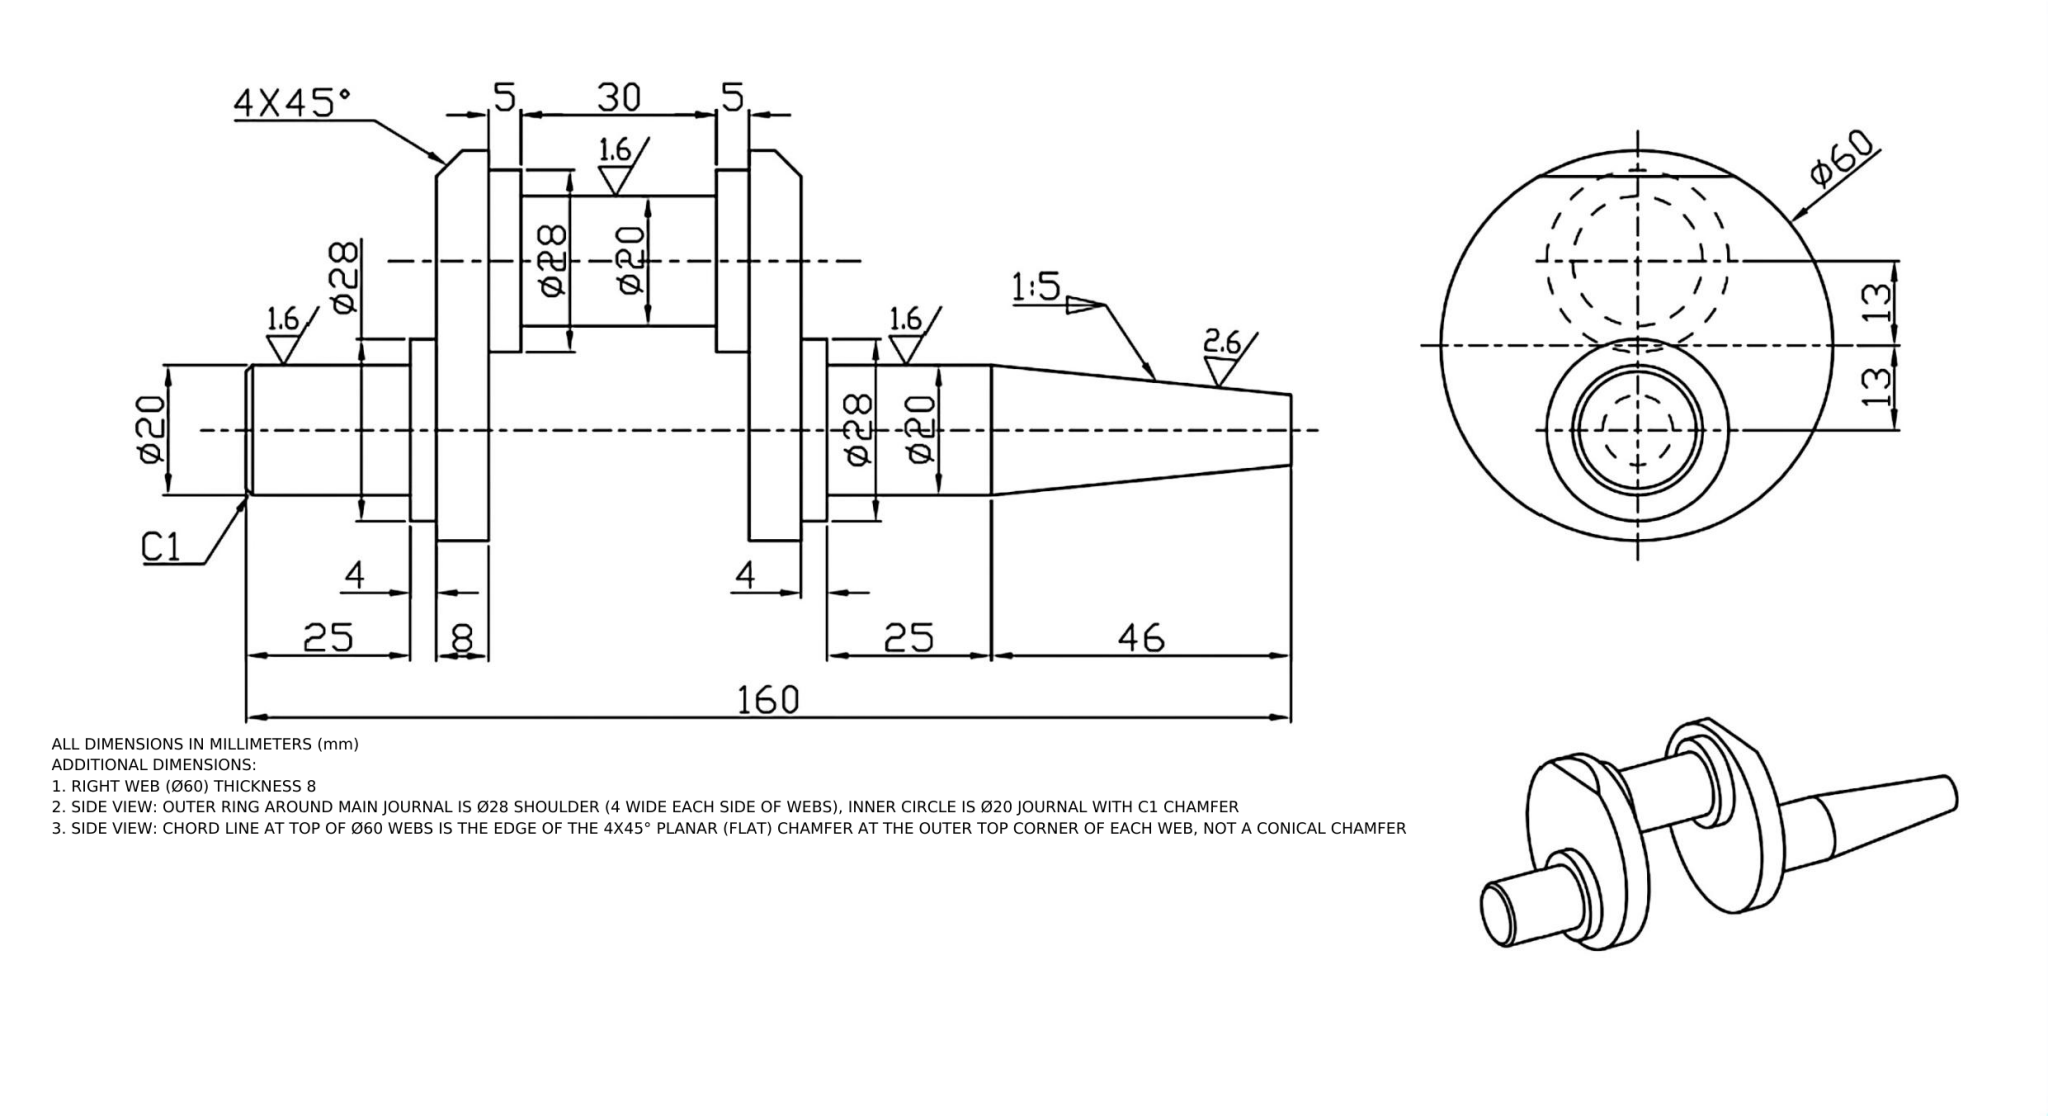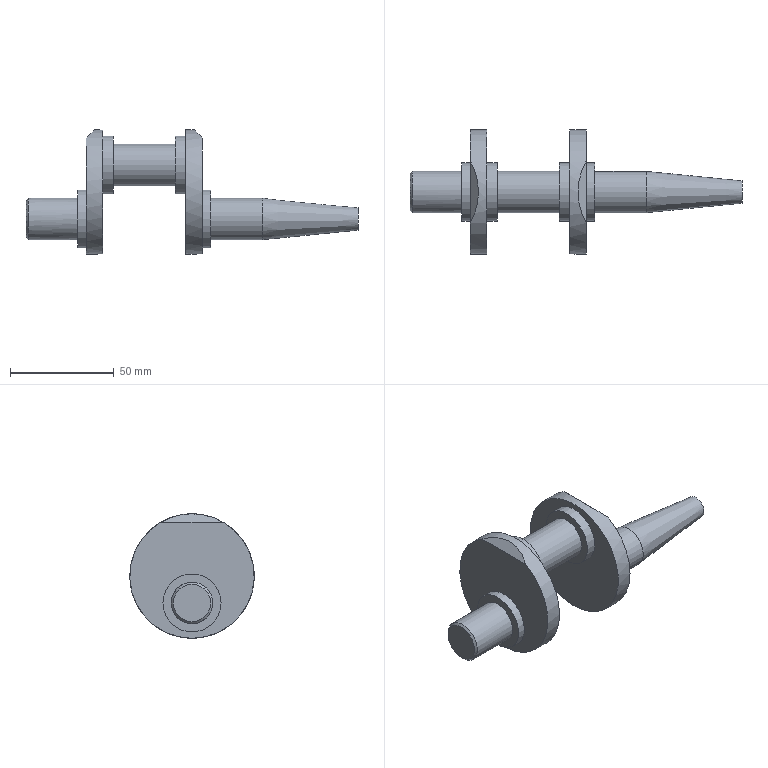Part | NX | mm | 1 solid | 23 faces | box 160 x 60 x 60 mm | volume 89987 mm3 | plane 12 | cylinder 9 | cone 2 | commonest cylinder face diameters 28 x4 20 x3 60 x2
STEP:
#1=CARTESIAN_POINT('',(0.,0.,0.));
#2=DIRECTION('',(0.,0.,1.));
#3=DIRECTION('',(1.,0.,0.));
#4=AXIS2_PLACEMENT_3D('',#1,#2,#3);
#5=(LENGTH_UNIT()NAMED_UNIT(*)SI_UNIT(.MILLI.,.METRE.));
#6=UNCERTAINTY_MEASURE_WITH_UNIT(LENGTH_MEASURE(0.00002),#5,'','');
#7=(NAMED_UNIT(*)PLANE_ANGLE_UNIT()SI_UNIT($,.RADIAN.));
#8=PLANE_ANGLE_MEASURE_WITH_UNIT(PLANE_ANGLE_MEASURE(0.01745),#7);
#9=DIMENSIONAL_EXPONENTS(0.,0.,0.,0.,0.,0.,0.);
#10=(CONVERSION_BASED_UNIT('',#8)NAMED_UNIT(#9)PLANE_ANGLE_UNIT());
#11=(NAMED_UNIT(*)SI_UNIT($,.STERADIAN.)SOLID_ANGLE_UNIT());
#12=(GEOMETRIC_REPRESENTATION_CONTEXT(3)GLOBAL_UNCERTAINTY_ASSIGNED_CONTEXT((#6))GLOBAL_UNIT_ASSIGNED_CONTEXT((#5,#10,#11))REPRESENTATION_CONTEXT('',''));
#13=SHAPE_REPRESENTATION('',(#4),#12);
#14=CARTESIAN_POINT('',(37.,30.,13.));
#15=VERTEX_POINT('',#14);
#16=CARTESIAN_POINT('',(37.,0.,13.));
#17=DIRECTION('',(1.,0.,0.));
#18=DIRECTION('',(0.,1.,-0.));
#19=AXIS2_PLACEMENT_3D('',#16,#17,#18);
#20=CIRCLE('',#19,30.);
#21=EDGE_CURVE('',#15,#15,#20,.T.);
#22=ORIENTED_EDGE('',*,*,#21,.F.);
#23=EDGE_LOOP('',(#22));
#24=FACE_BOUND('',#23,.T.);
#25=CARTESIAN_POINT('',(29.,-14.967,39.));
#26=VERTEX_POINT('',#25);
#27=CARTESIAN_POINT('',(29.,14.967,39.));
#28=VERTEX_POINT('',#27);
#29=CARTESIAN_POINT('',(3.,0.,13.));
#30=DIRECTION('',(-0.7071,0.,0.7071));
#31=DIRECTION('',(-0.7071,0.,-0.7071));
#32=AXIS2_PLACEMENT_3D('',#29,#30,#31);
#33=ELLIPSE('',#32,42.426,30.);
#34=EDGE_CURVE('',#26,#28,#33,.T.);
#35=ORIENTED_EDGE('',*,*,#34,.F.);
#36=CARTESIAN_POINT('',(29.,0.,13.));
#37=DIRECTION('',(1.,0.,0.));
#38=DIRECTION('',(0.,1.,-0.));
#39=AXIS2_PLACEMENT_3D('',#36,#37,#38);
#40=CIRCLE('',#39,30.);
#41=EDGE_CURVE('',#26,#28,#40,.T.);
#42=ORIENTED_EDGE('',*,*,#41,.T.);
#43=EDGE_LOOP('',(#35,#42));
#44=FACE_BOUND('',#43,.T.);
#45=CARTESIAN_POINT('',(37.,0.,13.));
#46=DIRECTION('',(-1.,0.,0.));
#47=DIRECTION('',(0.,0.,1.));
#48=AXIS2_PLACEMENT_3D('',#45,#46,#47);
#49=CYLINDRICAL_SURFACE('',#48,30.);
#50=ADVANCED_FACE('',(#24,#44),#49,.T.);
#51=CARTESIAN_POINT('',(1.,0.,-10.));
#52=VERTEX_POINT('',#51);
#53=CARTESIAN_POINT('',(1.,0.,0.));
#54=DIRECTION('',(1.,0.,0.));
#55=DIRECTION('',(0.,0.,-1.));
#56=AXIS2_PLACEMENT_3D('',#53,#54,#55);
#57=CIRCLE('',#56,10.);
#58=EDGE_CURVE('',#52,#52,#57,.T.);
#59=ORIENTED_EDGE('',*,*,#58,.T.);
#60=EDGE_LOOP('',(#59));
#61=FACE_BOUND('',#60,.T.);
#62=CARTESIAN_POINT('',(25.,10.,-0.));
#63=VERTEX_POINT('',#62);
#64=CARTESIAN_POINT('',(25.,0.,0.));
#65=DIRECTION('',(1.,0.,0.));
#66=DIRECTION('',(0.,1.,-0.));
#67=AXIS2_PLACEMENT_3D('',#64,#65,#66);
#68=CIRCLE('',#67,10.);
#69=EDGE_CURVE('',#63,#63,#68,.T.);
#70=ORIENTED_EDGE('',*,*,#69,.F.);
#71=EDGE_LOOP('',(#70));
#72=FACE_BOUND('',#71,.T.);
#73=CARTESIAN_POINT('',(25.,0.,0.));
#74=DIRECTION('',(-1.,0.,0.));
#75=DIRECTION('',(0.,0.,1.));
#76=AXIS2_PLACEMENT_3D('',#73,#74,#75);
#77=CYLINDRICAL_SURFACE('',#76,10.);
#78=ADVANCED_FACE('',(#61,#72),#77,.T.);
#79=CARTESIAN_POINT('',(0.,0.,-9.));
#80=VERTEX_POINT('',#79);
#81=CARTESIAN_POINT('',(0.,0.,0.));
#82=DIRECTION('',(-1.,0.,0.));
#83=DIRECTION('',(0.,0.,-1.));
#84=AXIS2_PLACEMENT_3D('',#81,#82,#83);
#85=CIRCLE('',#84,9.);
#86=EDGE_CURVE('',#80,#80,#85,.T.);
#87=ORIENTED_EDGE('',*,*,#86,.T.);
#88=EDGE_LOOP('',(#87));
#89=FACE_OUTER_BOUND('',#88,.T.);
#90=CARTESIAN_POINT('',(0.,0.,0.));
#91=DIRECTION('',(1.,0.,0.));
#92=DIRECTION('',(0.,0.,-1.));
#93=AXIS2_PLACEMENT_3D('',#90,#91,#92);
#94=PLANE('',#93);
#95=ADVANCED_FACE('',(#89),#94,.F.);
#96=ORIENTED_EDGE('',*,*,#86,.F.);
#97=EDGE_LOOP('',(#96));
#98=FACE_BOUND('',#97,.T.);
#99=ORIENTED_EDGE('',*,*,#58,.F.);
#100=EDGE_LOOP('',(#99));
#101=FACE_BOUND('',#100,.T.);
#102=CARTESIAN_POINT('',(1.,0.,0.));
#103=DIRECTION('',(1.,0.,0.));
#104=DIRECTION('',(-0.,0.,-1.));
#105=AXIS2_PLACEMENT_3D('',#102,#103,#104);
#106=CONICAL_SURFACE('',#105,10.,45.);
#107=ADVANCED_FACE('',(#98,#101),#106,.T.);
#108=CARTESIAN_POINT('',(37.,14.,26.));
#109=VERTEX_POINT('',#108);
#110=CARTESIAN_POINT('',(37.,0.,26.));
#111=DIRECTION('',(1.,0.,0.));
#112=DIRECTION('',(0.,1.,0.));
#113=AXIS2_PLACEMENT_3D('',#110,#111,#112);
#114=CIRCLE('',#113,14.);
#115=EDGE_CURVE('',#109,#109,#114,.T.);
#116=ORIENTED_EDGE('',*,*,#115,.F.);
#117=EDGE_LOOP('',(#116));
#118=FACE_BOUND('',#117,.T.);
#119=ORIENTED_EDGE('',*,*,#21,.T.);
#120=EDGE_LOOP('',(#119));
#121=FACE_BOUND('',#120,.T.);
#122=CARTESIAN_POINT('',(37.,0.,13.));
#123=DIRECTION('',(1.,0.,0.));
#124=DIRECTION('',(0.,0.,-1.));
#125=AXIS2_PLACEMENT_3D('',#122,#123,#124);
#126=PLANE('',#125);
#127=ADVANCED_FACE('',(#118,#121),#126,.T.);
#128=CARTESIAN_POINT('',(29.,14.,-0.));
#129=VERTEX_POINT('',#128);
#130=CARTESIAN_POINT('',(29.,0.,0.));
#131=DIRECTION('',(1.,0.,0.));
#132=DIRECTION('',(0.,1.,-0.));
#133=AXIS2_PLACEMENT_3D('',#130,#131,#132);
#134=CIRCLE('',#133,14.);
#135=EDGE_CURVE('',#129,#129,#134,.T.);
#136=ORIENTED_EDGE('',*,*,#135,.T.);
#137=EDGE_LOOP('',(#136));
#138=FACE_BOUND('',#137,.T.);
#139=ORIENTED_EDGE('',*,*,#41,.F.);
#140=CARTESIAN_POINT('',(29.,-47.,39.));
#141=DIRECTION('',(0.,1.,0.));
#142=VECTOR('',#141,1.);
#143=LINE('',#140,#142);
#144=EDGE_CURVE('',#26,#28,#143,.T.);
#145=ORIENTED_EDGE('',*,*,#144,.T.);
#146=EDGE_LOOP('',(#139,#145));
#147=FACE_BOUND('',#146,.T.);
#148=CARTESIAN_POINT('',(29.,0.,13.));
#149=DIRECTION('',(1.,0.,0.));
#150=DIRECTION('',(0.,0.,-1.));
#151=AXIS2_PLACEMENT_3D('',#148,#149,#150);
#152=PLANE('',#151);
#153=ADVANCED_FACE('',(#138,#147),#152,.F.);
#154=CARTESIAN_POINT('',(42.,14.,26.));
#155=VERTEX_POINT('',#154);
#156=CARTESIAN_POINT('',(42.,0.,26.));
#157=DIRECTION('',(1.,0.,0.));
#158=DIRECTION('',(0.,1.,0.));
#159=AXIS2_PLACEMENT_3D('',#156,#157,#158);
#160=CIRCLE('',#159,14.);
#161=EDGE_CURVE('',#155,#155,#160,.T.);
#162=ORIENTED_EDGE('',*,*,#161,.F.);
#163=EDGE_LOOP('',(#162));
#164=FACE_BOUND('',#163,.T.);
#165=ORIENTED_EDGE('',*,*,#115,.T.);
#166=EDGE_LOOP('',(#165));
#167=FACE_BOUND('',#166,.T.);
#168=CARTESIAN_POINT('',(42.,0.,26.));
#169=DIRECTION('',(-1.,0.,0.));
#170=DIRECTION('',(0.,0.,1.));
#171=AXIS2_PLACEMENT_3D('',#168,#169,#170);
#172=CYLINDRICAL_SURFACE('',#171,14.);
#173=ADVANCED_FACE('',(#164,#167),#172,.T.);
#174=CARTESIAN_POINT('',(42.,10.,26.));
#175=VERTEX_POINT('',#174);
#176=CARTESIAN_POINT('',(42.,0.,26.));
#177=DIRECTION('',(1.,0.,0.));
#178=DIRECTION('',(0.,1.,0.));
#179=AXIS2_PLACEMENT_3D('',#176,#177,#178);
#180=CIRCLE('',#179,10.);
#181=EDGE_CURVE('',#175,#175,#180,.T.);
#182=ORIENTED_EDGE('',*,*,#181,.F.);
#183=EDGE_LOOP('',(#182));
#184=FACE_BOUND('',#183,.T.);
#185=ORIENTED_EDGE('',*,*,#161,.T.);
#186=EDGE_LOOP('',(#185));
#187=FACE_BOUND('',#186,.T.);
#188=CARTESIAN_POINT('',(42.,0.,26.));
#189=DIRECTION('',(1.,0.,0.));
#190=DIRECTION('',(0.,0.,-1.));
#191=AXIS2_PLACEMENT_3D('',#188,#189,#190);
#192=PLANE('',#191);
#193=ADVANCED_FACE('',(#184,#187),#192,.T.);
#194=CARTESIAN_POINT('',(72.,10.,26.));
#195=VERTEX_POINT('',#194);
#196=CARTESIAN_POINT('',(72.,0.,26.));
#197=DIRECTION('',(1.,0.,0.));
#198=DIRECTION('',(0.,1.,0.));
#199=AXIS2_PLACEMENT_3D('',#196,#197,#198);
#200=CIRCLE('',#199,10.);
#201=EDGE_CURVE('',#195,#195,#200,.T.);
#202=ORIENTED_EDGE('',*,*,#201,.F.);
#203=EDGE_LOOP('',(#202));
#204=FACE_BOUND('',#203,.T.);
#205=ORIENTED_EDGE('',*,*,#181,.T.);
#206=EDGE_LOOP('',(#205));
#207=FACE_BOUND('',#206,.T.);
#208=CARTESIAN_POINT('',(72.,0.,26.));
#209=DIRECTION('',(-1.,0.,0.));
#210=DIRECTION('',(0.,0.,1.));
#211=AXIS2_PLACEMENT_3D('',#208,#209,#210);
#212=CYLINDRICAL_SURFACE('',#211,10.);
#213=ADVANCED_FACE('',(#204,#207),#212,.T.);
#214=CARTESIAN_POINT('',(85.,14.967,39.));
#215=VERTEX_POINT('',#214);
#216=CARTESIAN_POINT('',(85.,-14.967,39.));
#217=VERTEX_POINT('',#216);
#218=CARTESIAN_POINT('',(111.,0.,13.));
#219=DIRECTION('',(0.7071,0.,0.7071));
#220=DIRECTION('',(0.7071,0.,-0.7071));
#221=AXIS2_PLACEMENT_3D('',#218,#219,#220);
#222=ELLIPSE('',#221,42.426,30.);
#223=EDGE_CURVE('',#215,#217,#222,.T.);
#224=ORIENTED_EDGE('',*,*,#223,.F.);
#225=CARTESIAN_POINT('',(85.,0.,13.));
#226=DIRECTION('',(1.,0.,0.));
#227=DIRECTION('',(0.,1.,-0.));
#228=AXIS2_PLACEMENT_3D('',#225,#226,#227);
#229=CIRCLE('',#228,30.);
#230=EDGE_CURVE('',#217,#215,#229,.T.);
#231=ORIENTED_EDGE('',*,*,#230,.F.);
#232=EDGE_LOOP('',(#224,#231));
#233=FACE_BOUND('',#232,.T.);
#234=CARTESIAN_POINT('',(77.,30.,13.));
#235=VERTEX_POINT('',#234);
#236=CARTESIAN_POINT('',(77.,0.,13.));
#237=DIRECTION('',(1.,0.,0.));
#238=DIRECTION('',(0.,1.,-0.));
#239=AXIS2_PLACEMENT_3D('',#236,#237,#238);
#240=CIRCLE('',#239,30.);
#241=EDGE_CURVE('',#235,#235,#240,.T.);
#242=ORIENTED_EDGE('',*,*,#241,.T.);
#243=EDGE_LOOP('',(#242));
#244=FACE_BOUND('',#243,.T.);
#245=CARTESIAN_POINT('',(77.,0.,13.));
#246=DIRECTION('',(1.,0.,0.));
#247=DIRECTION('',(0.,0.,-1.));
#248=AXIS2_PLACEMENT_3D('',#245,#246,#247);
#249=CYLINDRICAL_SURFACE('',#248,30.);
#250=ADVANCED_FACE('',(#233,#244),#249,.T.);
#251=CARTESIAN_POINT('',(77.,14.,26.));
#252=VERTEX_POINT('',#251);
#253=CARTESIAN_POINT('',(77.,0.,26.));
#254=DIRECTION('',(1.,0.,0.));
#255=DIRECTION('',(0.,1.,0.));
#256=AXIS2_PLACEMENT_3D('',#253,#254,#255);
#257=CIRCLE('',#256,14.);
#258=EDGE_CURVE('',#252,#252,#257,.T.);
#259=ORIENTED_EDGE('',*,*,#258,.T.);
#260=EDGE_LOOP('',(#259));
#261=FACE_BOUND('',#260,.T.);
#262=ORIENTED_EDGE('',*,*,#241,.F.);
#263=EDGE_LOOP('',(#262));
#264=FACE_BOUND('',#263,.T.);
#265=CARTESIAN_POINT('',(77.,0.,13.));
#266=DIRECTION('',(1.,0.,0.));
#267=DIRECTION('',(0.,0.,-1.));
#268=AXIS2_PLACEMENT_3D('',#265,#266,#267);
#269=PLANE('',#268);
#270=ADVANCED_FACE('',(#261,#264),#269,.F.);
#271=CARTESIAN_POINT('',(85.,-47.,39.));
#272=DIRECTION('',(0.,1.,0.));
#273=VECTOR('',#272,1.);
#274=LINE('',#271,#273);
#275=EDGE_CURVE('',#217,#215,#274,.T.);
#276=ORIENTED_EDGE('',*,*,#275,.F.);
#277=ORIENTED_EDGE('',*,*,#230,.T.);
#278=EDGE_LOOP('',(#276,#277));
#279=FACE_BOUND('',#278,.T.);
#280=CARTESIAN_POINT('',(85.,14.,-0.));
#281=VERTEX_POINT('',#280);
#282=CARTESIAN_POINT('',(85.,0.,0.));
#283=DIRECTION('',(1.,0.,0.));
#284=DIRECTION('',(0.,1.,-0.));
#285=AXIS2_PLACEMENT_3D('',#282,#283,#284);
#286=CIRCLE('',#285,14.);
#287=EDGE_CURVE('',#281,#281,#286,.T.);
#288=ORIENTED_EDGE('',*,*,#287,.F.);
#289=EDGE_LOOP('',(#288));
#290=FACE_BOUND('',#289,.T.);
#291=CARTESIAN_POINT('',(85.,0.,13.));
#292=DIRECTION('',(1.,0.,0.));
#293=DIRECTION('',(0.,0.,-1.));
#294=AXIS2_PLACEMENT_3D('',#291,#292,#293);
#295=PLANE('',#294);
#296=ADVANCED_FACE('',(#279,#290),#295,.T.);
#297=CARTESIAN_POINT('',(72.,14.,26.));
#298=VERTEX_POINT('',#297);
#299=CARTESIAN_POINT('',(72.,0.,26.));
#300=DIRECTION('',(1.,0.,0.));
#301=DIRECTION('',(0.,1.,0.));
#302=AXIS2_PLACEMENT_3D('',#299,#300,#301);
#303=CIRCLE('',#302,14.);
#304=EDGE_CURVE('',#298,#298,#303,.T.);
#305=ORIENTED_EDGE('',*,*,#304,.T.);
#306=EDGE_LOOP('',(#305));
#307=FACE_BOUND('',#306,.T.);
#308=ORIENTED_EDGE('',*,*,#258,.F.);
#309=EDGE_LOOP('',(#308));
#310=FACE_BOUND('',#309,.T.);
#311=CARTESIAN_POINT('',(72.,0.,26.));
#312=DIRECTION('',(1.,0.,0.));
#313=DIRECTION('',(0.,0.,-1.));
#314=AXIS2_PLACEMENT_3D('',#311,#312,#313);
#315=CYLINDRICAL_SURFACE('',#314,14.);
#316=ADVANCED_FACE('',(#307,#310),#315,.T.);
#317=ORIENTED_EDGE('',*,*,#201,.T.);
#318=EDGE_LOOP('',(#317));
#319=FACE_BOUND('',#318,.T.);
#320=ORIENTED_EDGE('',*,*,#304,.F.);
#321=EDGE_LOOP('',(#320));
#322=FACE_BOUND('',#321,.T.);
#323=CARTESIAN_POINT('',(72.,0.,26.));
#324=DIRECTION('',(1.,0.,0.));
#325=DIRECTION('',(0.,0.,-1.));
#326=AXIS2_PLACEMENT_3D('',#323,#324,#325);
#327=PLANE('',#326);
#328=ADVANCED_FACE('',(#319,#322),#327,.F.);
#329=ORIENTED_EDGE('',*,*,#287,.T.);
#330=EDGE_LOOP('',(#329));
#331=FACE_BOUND('',#330,.T.);
#332=CARTESIAN_POINT('',(89.,14.,-0.));
#333=VERTEX_POINT('',#332);
#334=CARTESIAN_POINT('',(89.,0.,0.));
#335=DIRECTION('',(1.,0.,0.));
#336=DIRECTION('',(0.,1.,-0.));
#337=AXIS2_PLACEMENT_3D('',#334,#335,#336);
#338=CIRCLE('',#337,14.);
#339=EDGE_CURVE('',#333,#333,#338,.T.);
#340=ORIENTED_EDGE('',*,*,#339,.F.);
#341=EDGE_LOOP('',(#340));
#342=FACE_BOUND('',#341,.T.);
#343=CARTESIAN_POINT('',(85.,0.,0.));
#344=DIRECTION('',(1.,0.,0.));
#345=DIRECTION('',(0.,0.,-1.));
#346=AXIS2_PLACEMENT_3D('',#343,#344,#345);
#347=CYLINDRICAL_SURFACE('',#346,14.);
#348=ADVANCED_FACE('',(#331,#342),#347,.T.);
#349=CARTESIAN_POINT('',(89.,0.,-10.));
#350=VERTEX_POINT('',#349);
#351=CARTESIAN_POINT('',(89.,0.,-0.));
#352=DIRECTION('',(1.,0.,0.));
#353=DIRECTION('',(0.,0.,-1.));
#354=AXIS2_PLACEMENT_3D('',#351,#352,#353);
#355=CIRCLE('',#354,10.);
#356=EDGE_CURVE('',#350,#350,#355,.T.);
#357=ORIENTED_EDGE('',*,*,#356,.F.);
#358=EDGE_LOOP('',(#357));
#359=FACE_BOUND('',#358,.T.);
#360=ORIENTED_EDGE('',*,*,#339,.T.);
#361=EDGE_LOOP('',(#360));
#362=FACE_BOUND('',#361,.T.);
#363=CARTESIAN_POINT('',(89.,0.,0.));
#364=DIRECTION('',(1.,0.,0.));
#365=DIRECTION('',(0.,0.,-1.));
#366=AXIS2_PLACEMENT_3D('',#363,#364,#365);
#367=PLANE('',#366);
#368=ADVANCED_FACE('',(#359,#362),#367,.T.);
#369=CARTESIAN_POINT('',(160.,0.,-5.4));
#370=VERTEX_POINT('',#369);
#371=CARTESIAN_POINT('',(160.,0.,0.));
#372=DIRECTION('',(1.,0.,0.));
#373=DIRECTION('',(0.,0.,-1.));
#374=AXIS2_PLACEMENT_3D('',#371,#372,#373);
#375=CIRCLE('',#374,5.4);
#376=EDGE_CURVE('',#370,#370,#375,.T.);
#377=ORIENTED_EDGE('',*,*,#376,.T.);
#378=EDGE_LOOP('',(#377));
#379=FACE_OUTER_BOUND('',#378,.T.);
#380=CARTESIAN_POINT('',(160.,0.,0.));
#381=DIRECTION('',(1.,0.,0.));
#382=DIRECTION('',(0.,0.,-1.));
#383=AXIS2_PLACEMENT_3D('',#380,#381,#382);
#384=PLANE('',#383);
#385=ADVANCED_FACE('',(#379),#384,.T.);
#386=CARTESIAN_POINT('',(114.,0.,-10.));
#387=VERTEX_POINT('',#386);
#388=CARTESIAN_POINT('',(114.,0.,-0.));
#389=DIRECTION('',(1.,0.,0.));
#390=DIRECTION('',(0.,0.,-1.));
#391=AXIS2_PLACEMENT_3D('',#388,#389,#390);
#392=CIRCLE('',#391,10.);
#393=EDGE_CURVE('',#387,#387,#392,.T.);
#394=ORIENTED_EDGE('',*,*,#393,.T.);
#395=EDGE_LOOP('',(#394));
#396=FACE_BOUND('',#395,.T.);
#397=ORIENTED_EDGE('',*,*,#376,.F.);
#398=EDGE_LOOP('',(#397));
#399=FACE_BOUND('',#398,.T.);
#400=CARTESIAN_POINT('',(160.,0.,0.));
#401=DIRECTION('',(-1.,0.,-0.));
#402=DIRECTION('',(0.,0.,1.));
#403=AXIS2_PLACEMENT_3D('',#400,#401,#402);
#404=CONICAL_SURFACE('',#403,5.4,5.711);
#405=ADVANCED_FACE('',(#396,#399),#404,.T.);
#406=ORIENTED_EDGE('',*,*,#356,.T.);
#407=EDGE_LOOP('',(#406));
#408=FACE_BOUND('',#407,.T.);
#409=ORIENTED_EDGE('',*,*,#393,.F.);
#410=EDGE_LOOP('',(#409));
#411=FACE_BOUND('',#410,.T.);
#412=CARTESIAN_POINT('',(89.,0.,-0.));
#413=DIRECTION('',(1.,0.,0.));
#414=DIRECTION('',(0.,0.,-1.));
#415=AXIS2_PLACEMENT_3D('',#412,#413,#414);
#416=CYLINDRICAL_SURFACE('',#415,10.);
#417=ADVANCED_FACE('',(#408,#411),#416,.T.);
#418=ORIENTED_EDGE('',*,*,#135,.F.);
#419=EDGE_LOOP('',(#418));
#420=FACE_BOUND('',#419,.T.);
#421=CARTESIAN_POINT('',(25.,14.,-0.));
#422=VERTEX_POINT('',#421);
#423=CARTESIAN_POINT('',(25.,0.,0.));
#424=DIRECTION('',(1.,0.,0.));
#425=DIRECTION('',(0.,1.,-0.));
#426=AXIS2_PLACEMENT_3D('',#423,#424,#425);
#427=CIRCLE('',#426,14.);
#428=EDGE_CURVE('',#422,#422,#427,.T.);
#429=ORIENTED_EDGE('',*,*,#428,.T.);
#430=EDGE_LOOP('',(#429));
#431=FACE_BOUND('',#430,.T.);
#432=CARTESIAN_POINT('',(29.,0.,0.));
#433=DIRECTION('',(-1.,0.,0.));
#434=DIRECTION('',(0.,0.,1.));
#435=AXIS2_PLACEMENT_3D('',#432,#433,#434);
#436=CYLINDRICAL_SURFACE('',#435,14.);
#437=ADVANCED_FACE('',(#420,#431),#436,.T.);
#438=ORIENTED_EDGE('',*,*,#69,.T.);
#439=EDGE_LOOP('',(#438));
#440=FACE_BOUND('',#439,.T.);
#441=ORIENTED_EDGE('',*,*,#428,.F.);
#442=EDGE_LOOP('',(#441));
#443=FACE_BOUND('',#442,.T.);
#444=CARTESIAN_POINT('',(25.,0.,0.));
#445=DIRECTION('',(1.,0.,0.));
#446=DIRECTION('',(0.,0.,-1.));
#447=AXIS2_PLACEMENT_3D('',#444,#445,#446);
#448=PLANE('',#447);
#449=ADVANCED_FACE('',(#440,#443),#448,.F.);
#450=ORIENTED_EDGE('',*,*,#34,.T.);
#451=ORIENTED_EDGE('',*,*,#144,.F.);
#452=EDGE_LOOP('',(#450,#451));
#453=FACE_OUTER_BOUND('',#452,.T.);
#454=CARTESIAN_POINT('',(29.,-47.,39.));
#455=DIRECTION('',(-0.7071,0.,0.7071));
#456=DIRECTION('',(0.7071,0.,0.7071));
#457=AXIS2_PLACEMENT_3D('',#454,#455,#456);
#458=PLANE('',#457);
#459=ADVANCED_FACE('',(#453),#458,.T.);
#460=ORIENTED_EDGE('',*,*,#223,.T.);
#461=ORIENTED_EDGE('',*,*,#275,.T.);
#462=EDGE_LOOP('',(#460,#461));
#463=FACE_OUTER_BOUND('',#462,.T.);
#464=CARTESIAN_POINT('',(85.,-47.,39.));
#465=DIRECTION('',(-0.7071,0.,-0.7071));
#466=DIRECTION('',(-0.7071,0.,0.7071));
#467=AXIS2_PLACEMENT_3D('',#464,#465,#466);
#468=PLANE('',#467);
#469=ADVANCED_FACE('',(#463),#468,.F.);
#470=CLOSED_SHELL('',(#50,#78,#95,#107,#127,#153,#173,#193,#213,#250,#270,#296,#316,#328,#348,#368,#385,#405,#417,#437,#449,#459,#469));
#471=MANIFOLD_SOLID_BREP('',#470);
#472=ADVANCED_BREP_SHAPE_REPRESENTATION('',(#471),#12);
#473=SHAPE_REPRESENTATION_RELATIONSHIP('','',#13,#472);
#474=PRESENTATION_LAYER_ASSIGNMENT('','',(#471));
#475=COLOUR_RGB('',1.,0.6,0.);
#476=FILL_AREA_STYLE_COLOUR('',#475);
#477=FILL_AREA_STYLE('',(#476));
#478=SURFACE_STYLE_FILL_AREA(#477);
#479=SURFACE_SIDE_STYLE('',(#478));
#480=SURFACE_STYLE_USAGE(.BOTH.,#479);
#481=PRESENTATION_STYLE_ASSIGNMENT((#480));
#482=STYLED_ITEM('',(#481),#471);
#483=MECHANICAL_DESIGN_GEOMETRIC_PRESENTATION_REPRESENTATION('',(#482),#12);